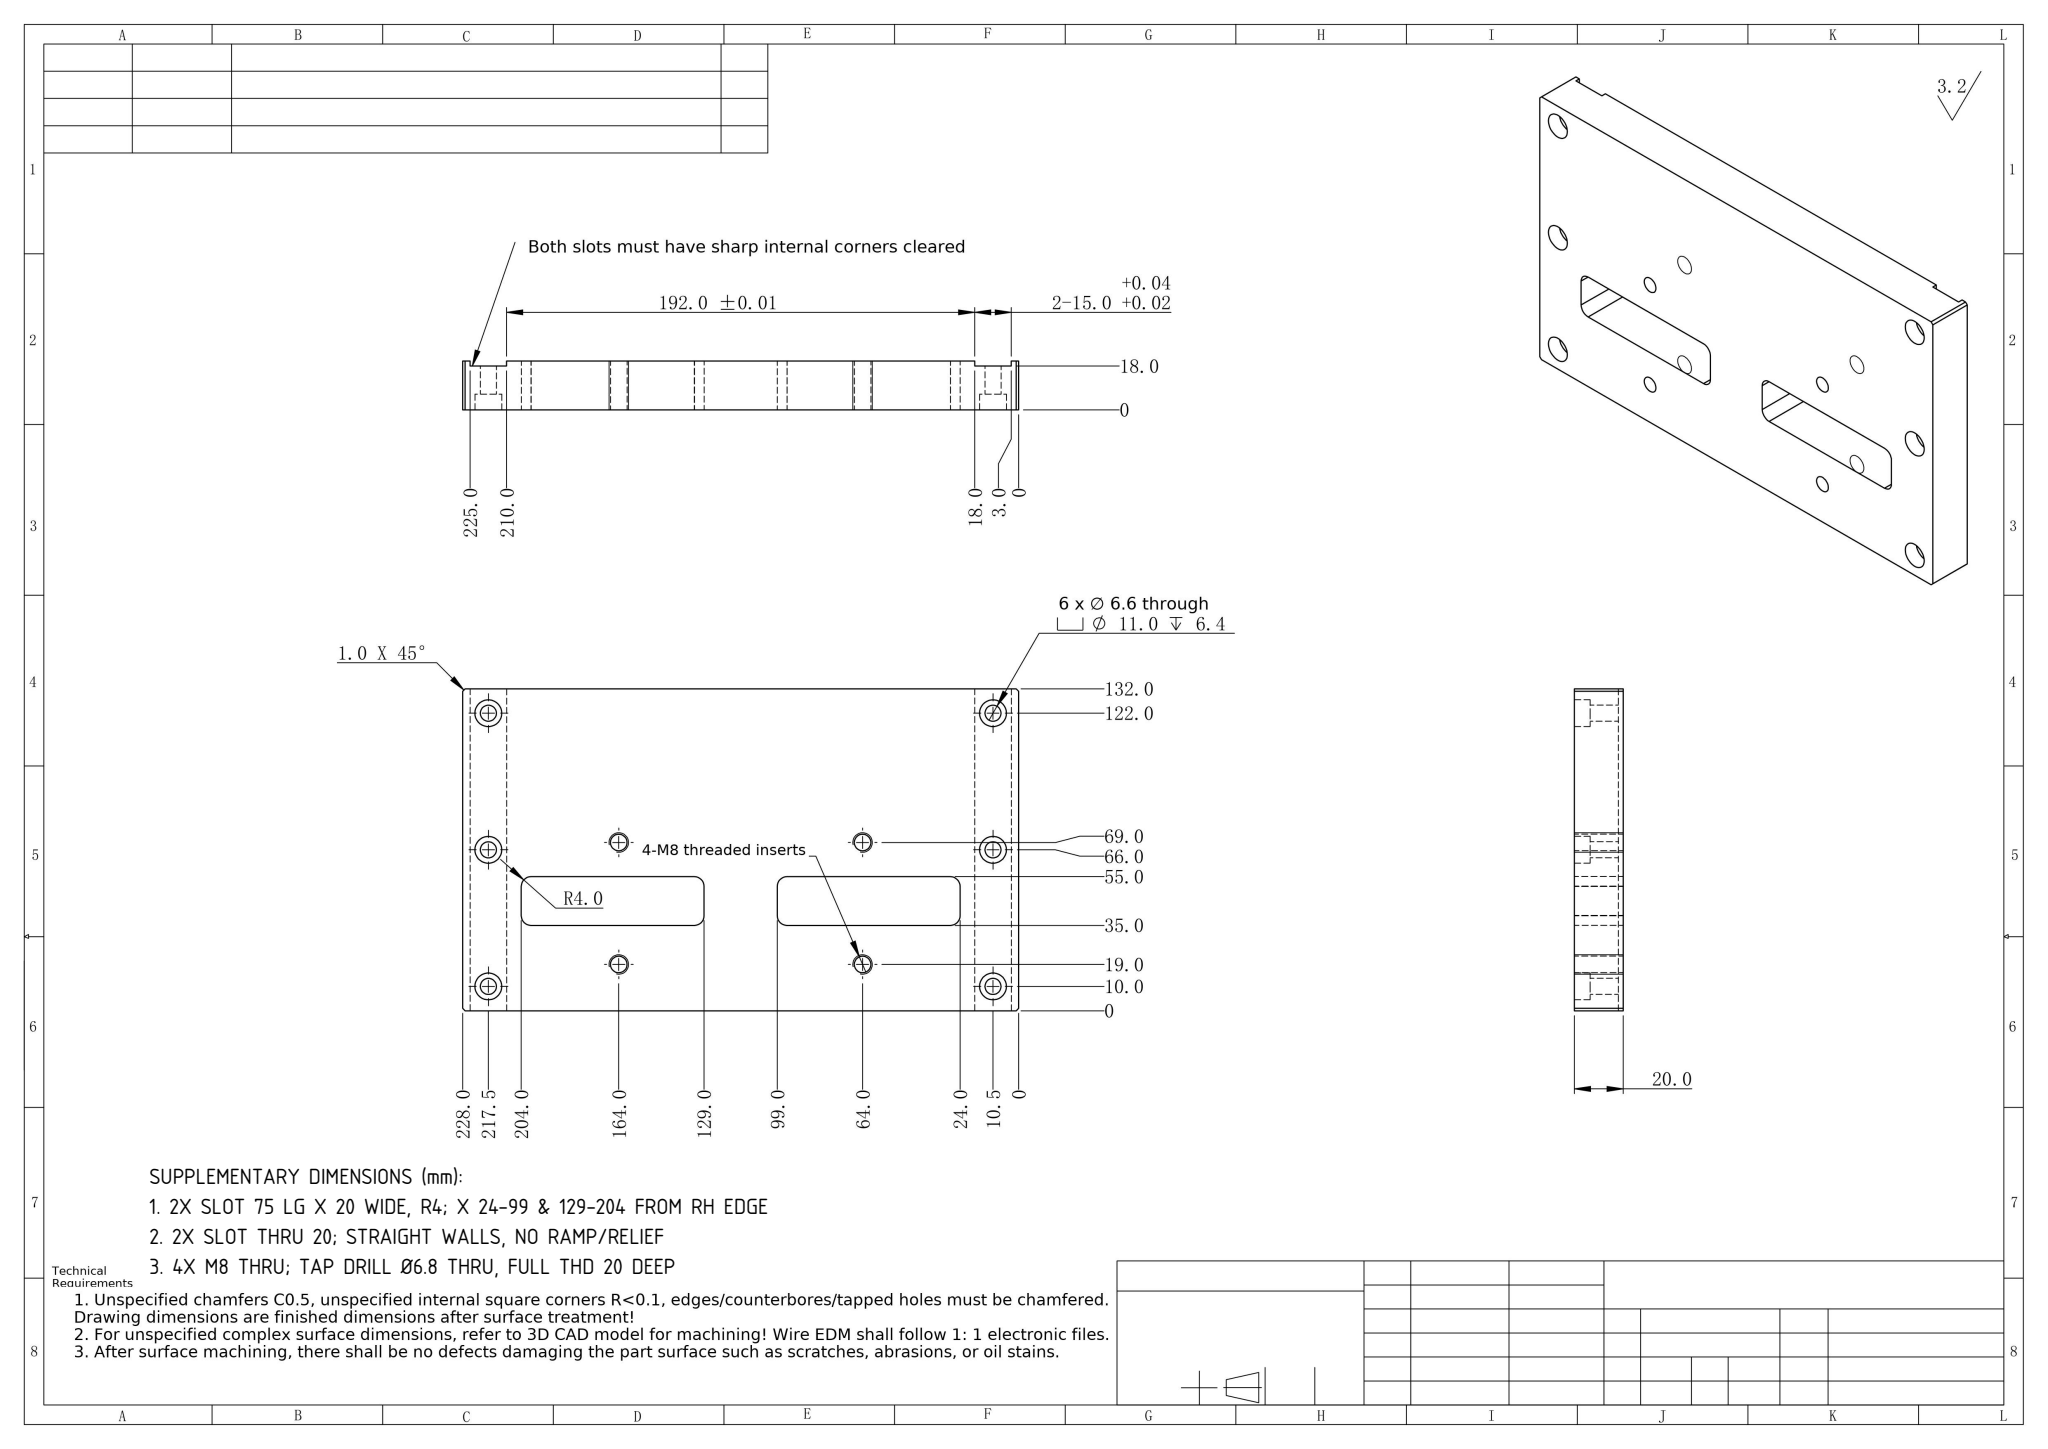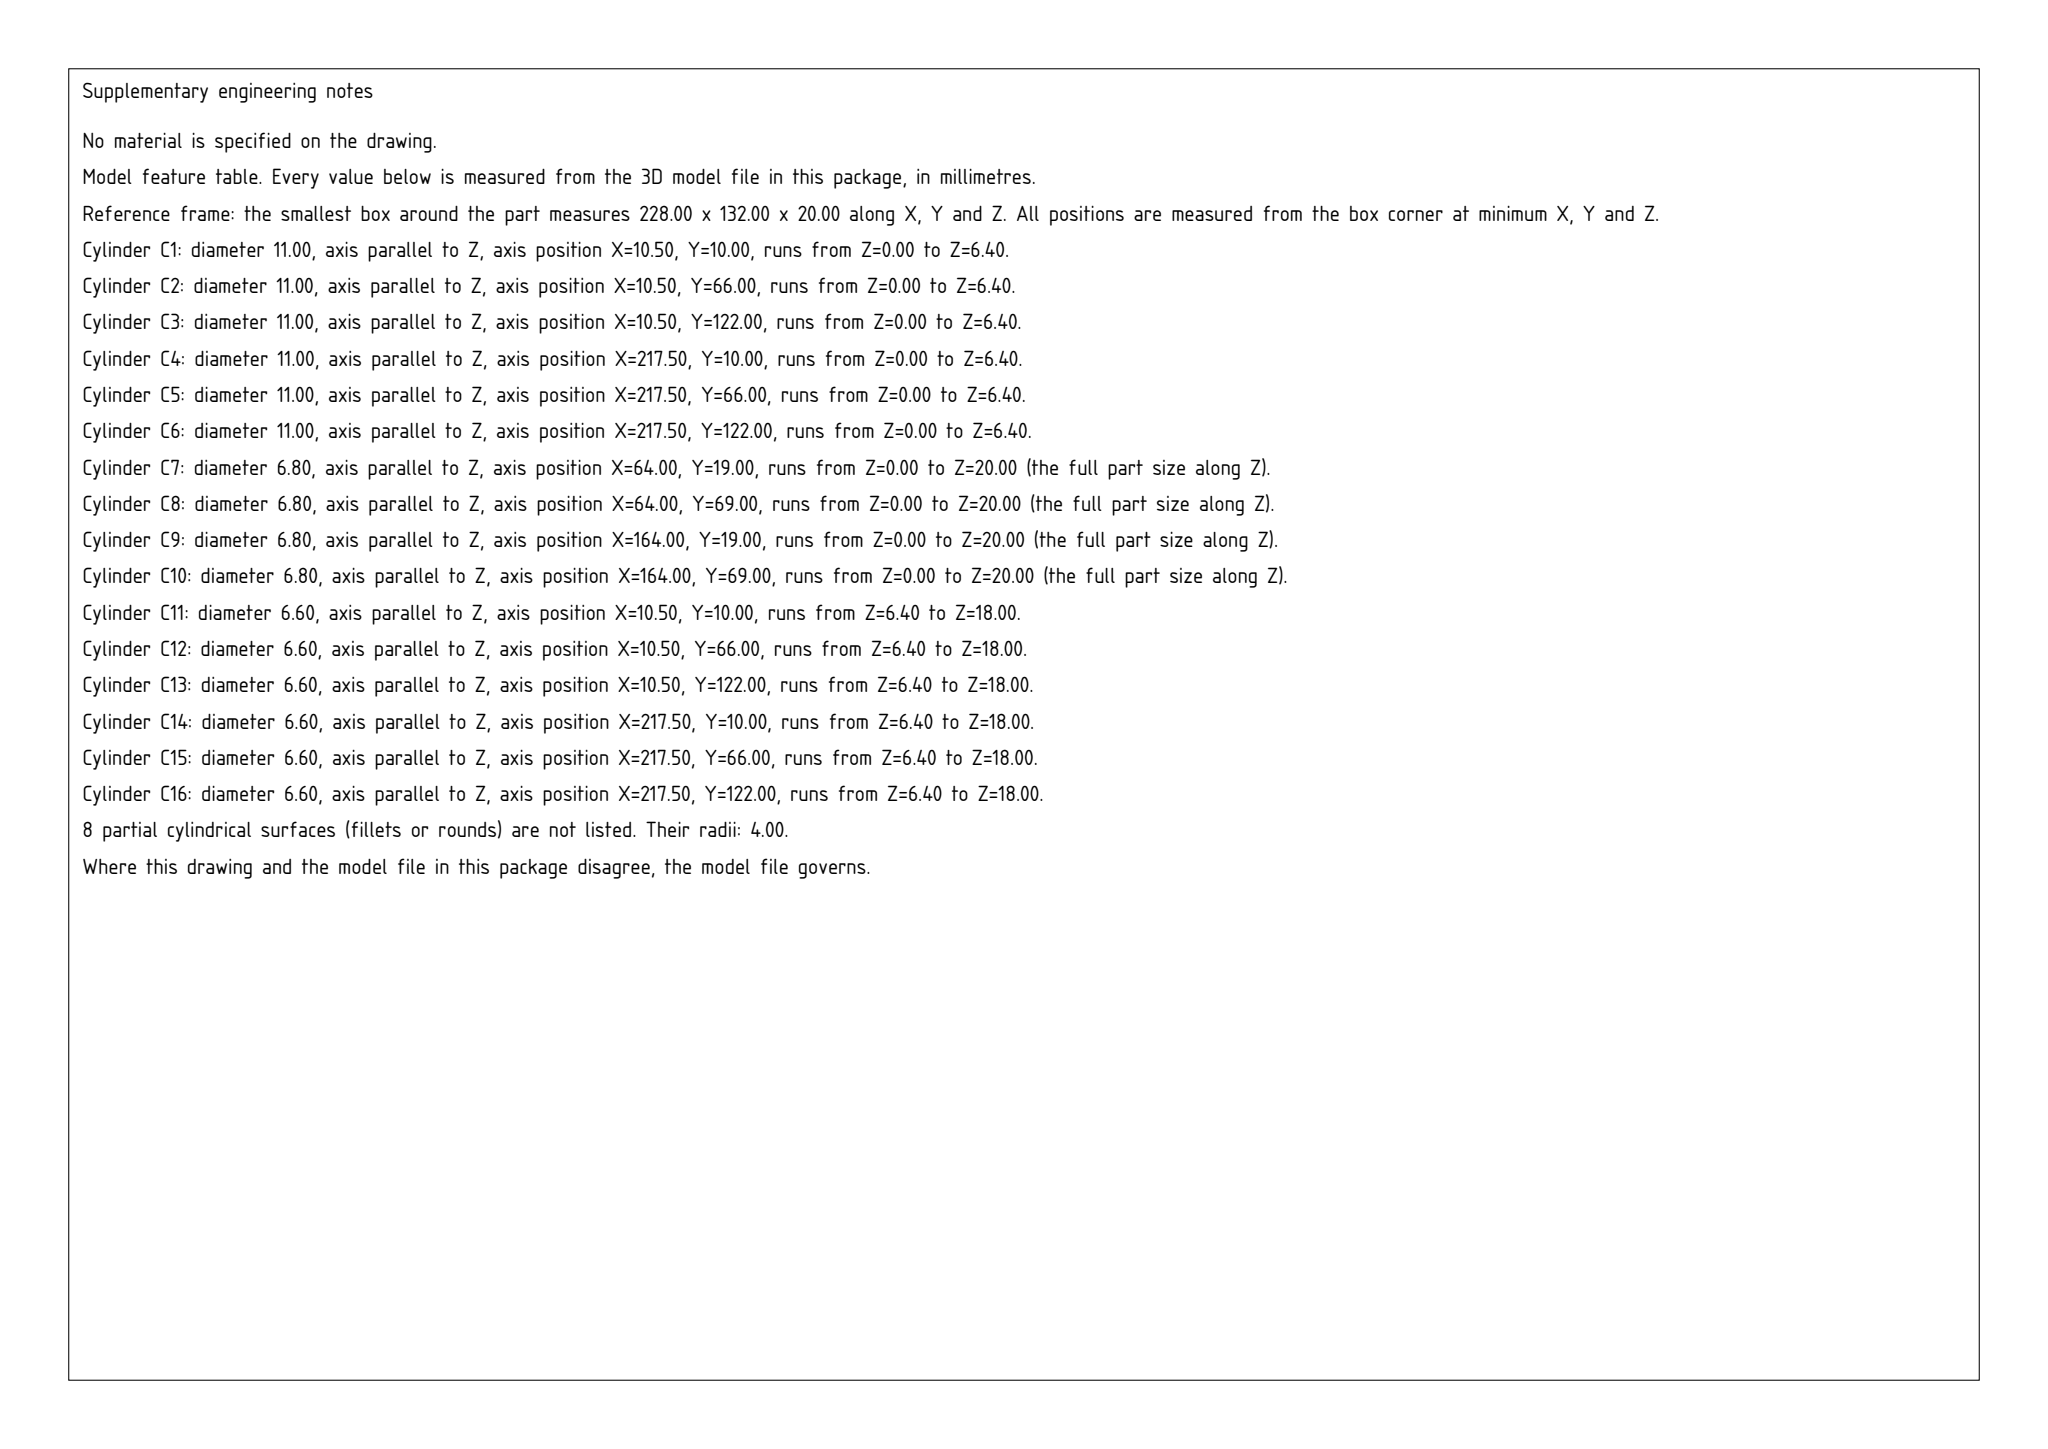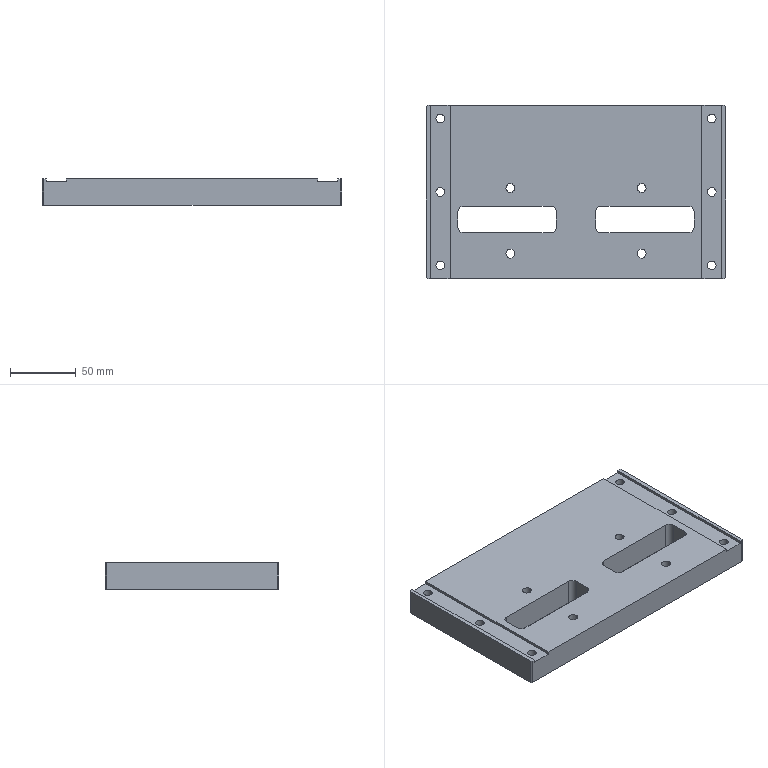Part | SolidWorks | mm | 1 solid | 72 faces | box 228 x 132 x 20 mm | volume 525574 mm3 | cylinder 40 | plane 32 | commonest cylinder face diameters 11 x12 6.6 x12 6.8 x8 8 x8
build123d program:
from build123d import *

# Parameters (mm, degrees)
SKETCH1_W                                       = 228
SKETCH1_H                                       = 132
BOSS_EXTRUDE1_DEPTH                             = 10
M8_TAPPED_HOLE1_D                               = 6.8
SKETCH4_W                                       = 15
SKETCH4_H                                       = 132
CUT_EXTRUDE1_DEPTH                              = 2
M6_HEX_SOCKET_HEAD_CAP_SCREW_CBORE1_D           = 6.6
M6_HEX_SOCKET_HEAD_CAP_SCREW_CBORE1_CBORE_D     = 11
M6_HEX_SOCKET_HEAD_CAP_SCREW_CBORE1_CBORE_DEPTH = 6.4
CHAMFER1_SIZE                                   = 1
SKETCH7_W                                       = 75
SKETCH7_H                                       = 20
CUT_EXTRUDE2_DEPTH                              = 265.212
FILLET1_R                                       = 4


with BuildPart() as part:
    # Sketch1 → Boss-Extrude1 (new, symmetric)
    with BuildSketch(Plane.XY):
        with Locations((114, 66)):
            Rectangle(SKETCH1_W, SKETCH1_H)
    extrude(amount=BOSS_EXTRUDE1_DEPTH, both=True)

    # M8 Tapped Hole1 (through all)
    with Locations(Plane.XY.offset(10)):
        with Locations((64, 19), (164, 19), (64, 69), (164, 69)):
            Hole(M8_TAPPED_HOLE1_D / 2)

    # Sketch4 → Cut-Extrude1 (cut)
    with BuildSketch(Plane.XY.offset(10)):
        with Locations((10.5, 66)):
            Rectangle(SKETCH4_W, SKETCH4_H)
        with Locations((217.5, 66)):
            Rectangle(SKETCH4_W, SKETCH4_H)
    extrude(amount=-CUT_EXTRUDE1_DEPTH, mode=Mode.SUBTRACT)

    # M6 Hex Socket Head Cap Screw CBORE1 (through all)
    with Locations(Plane(origin=(0, 0, -10), x_dir=(-1, 0, 0), z_dir=(0, 0, -1))):
        with Locations((-217.5, 122), (-217.5, 66), (-217.5, 10), (-10.5, 122), (-10.5, 66), (-10.5, 10)):
            CounterBoreHole(M6_HEX_SOCKET_HEAD_CAP_SCREW_CBORE1_D / 2, M6_HEX_SOCKET_HEAD_CAP_SCREW_CBORE1_CBORE_D / 2, M6_HEX_SOCKET_HEAD_CAP_SCREW_CBORE1_CBORE_DEPTH)

    # Chamfer1
    chamfer1_edges = [part.edges().sort_by_distance(p)[0] for p in [
        (0, 132, 0),
        (228, 132, 0),
        (228, 0, 0),
        (0, 0, 0),
    ]]
    chamfer(chamfer1_edges, length=CHAMFER1_SIZE)

    # Sketch7 → Cut-Extrude2 (cut, through all)
    with BuildSketch(Plane(origin=(0, 0, -10), x_dir=(-1, 0, 0), z_dir=(0, 0, -1))):
        with Locations((-166.5, 45)):
            Rectangle(SKETCH7_W, SKETCH7_H)
        with Locations((-61.5, 45)):
            Rectangle(SKETCH7_W, SKETCH7_H)
    extrude(amount=-CUT_EXTRUDE2_DEPTH, mode=Mode.SUBTRACT)

    # Fillet1
    fillet1_edges = [part.edges().sort_by_distance(p)[0] for p in [
        (204, 35, 0),
        (204, 55, 0),
        (129, 55, 0),
        (129, 35, 0),
        (99, 35, 0),
        (99, 55, 0),
        (24, 55, 0),
        (24, 35, 0),
    ]]
    fillet(fillet1_edges, radius=FILLET1_R)


solid = part.part